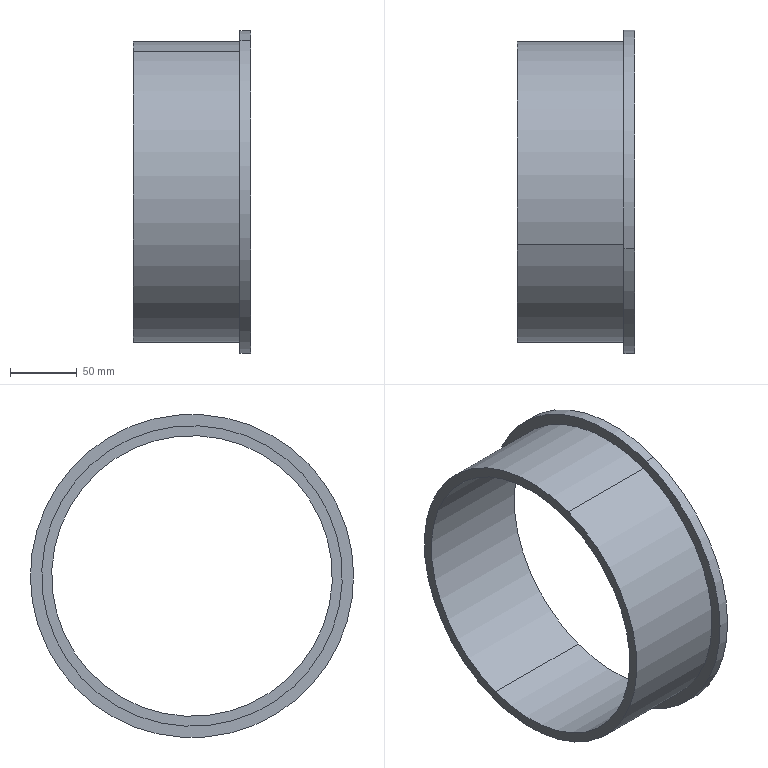Component | SolidWorks | AdjustingScrew-1 | 1 solid | 9 faces | box 88 x 243 x 243 mm | volume 503145 mm3 | cylinder 6 | plane 3 | commonest cylinder face diameters 226 x2 243 x2 211 x2
build123d program:
from build123d import *


with BuildPart() as part:
    # Sketch1 → Revolve1 (revolve)
    with BuildSketch(Plane.XY, mode=Mode.PRIVATE) as revolve1_sk:
        Polygon((0, 105.5), (88, 105.5), (88, 121.5), (80, 121.5), (80, 113), (0, 113), align=None)
    revolve(revolve1_sk.sketch.rotate(Axis((0, 0, 0), (1, 0, 0)), 90), axis=Axis((0, 0, 0), (1, 0, 0)))


solid = part.part

# Placed as in the assembly
solid = solid.moved(Location((-126, 0, 0), (0, 0, 0)))
STEP:
#1=COLOUR_RGB('',0.7922,0.8196,0.9333);
#2=FILL_AREA_STYLE_COLOUR('',#1);
#3=FILL_AREA_STYLE('',(#2));
#4=SURFACE_STYLE_FILL_AREA(#3);
#5=SURFACE_SIDE_STYLE('',(#4));
#6=SURFACE_STYLE_USAGE(.BOTH.,#5);
#7=PRESENTATION_STYLE_ASSIGNMENT((#6));
#8=CARTESIAN_POINT('',(-1.811,-1.573,4.161));
#9=VERTEX_POINT('',#8);
#10=CARTESIAN_POINT('',(-1.811,1.573,-4.161));
#11=VERTEX_POINT('',#10);
#12=CARTESIAN_POINT('',(-1.811,-0.,0.));
#13=DIRECTION('',(-1.,-0.,0.));
#14=DIRECTION('',(0.,-0.3537,0.9354));
#15=AXIS2_PLACEMENT_3D('',#12,#13,#14);
#16=CIRCLE('',#15,4.449);
#17=EDGE_CURVE('',#9,#11,#16,.T.);
#18=ORIENTED_EDGE('',*,*,#17,.T.);
#19=CARTESIAN_POINT('',(-4.961,1.573,-4.161));
#20=VERTEX_POINT('',#19);
#21=CARTESIAN_POINT('',(-4.961,1.573,-4.161));
#22=DIRECTION('',(-1.,-0.,0.));
#23=VECTOR('',#22,39.37);
#24=LINE('',#21,#23);
#25=EDGE_CURVE('',#11,#20,#24,.T.);
#26=ORIENTED_EDGE('',*,*,#25,.T.);
#27=CARTESIAN_POINT('',(-4.961,-1.573,4.161));
#28=VERTEX_POINT('',#27);
#29=CARTESIAN_POINT('',(-4.961,-0.,0.));
#30=DIRECTION('',(-1.,-0.,0.));
#31=DIRECTION('',(0.,-0.3537,0.9354));
#32=AXIS2_PLACEMENT_3D('',#29,#30,#31);
#33=CIRCLE('',#32,4.449);
#34=EDGE_CURVE('',#28,#20,#33,.T.);
#35=ORIENTED_EDGE('',*,*,#34,.F.);
#36=CARTESIAN_POINT('',(-4.961,-1.573,4.161));
#37=DIRECTION('',(-1.,-0.,0.));
#38=VECTOR('',#37,39.37);
#39=LINE('',#36,#38);
#40=EDGE_CURVE('',#9,#28,#39,.T.);
#41=ORIENTED_EDGE('',*,*,#40,.F.);
#42=EDGE_LOOP('',(#18,#26,#35,#41));
#43=FACE_OUTER_BOUND('',#42,.T.);
#44=CARTESIAN_POINT('',(-4.961,-0.,0.));
#45=DIRECTION('',(-1.,-0.,0.));
#46=DIRECTION('',(0.,-0.3537,0.9354));
#47=AXIS2_PLACEMENT_3D('',#44,#45,#46);
#48=CYLINDRICAL_SURFACE('',#47,4.449);
#49=ADVANCED_FACE('',(#43),#48,.T.);
#50=CARTESIAN_POINT('',(-1.496,-1.692,4.474));
#51=VERTEX_POINT('',#50);
#52=CARTESIAN_POINT('',(-1.496,1.692,-4.474));
#53=VERTEX_POINT('',#52);
#54=CARTESIAN_POINT('',(-1.496,-0.,0.));
#55=DIRECTION('',(-1.,-0.,0.));
#56=DIRECTION('',(0.,-0.3537,0.9354));
#57=AXIS2_PLACEMENT_3D('',#54,#55,#56);
#58=CIRCLE('',#57,4.783);
#59=EDGE_CURVE('',#51,#53,#58,.T.);
#60=ORIENTED_EDGE('',*,*,#59,.T.);
#61=CARTESIAN_POINT('',(-1.811,1.692,-4.474));
#62=VERTEX_POINT('',#61);
#63=CARTESIAN_POINT('',(-4.961,1.692,-4.474));
#64=DIRECTION('',(-1.,-0.,0.));
#65=VECTOR('',#64,39.37);
#66=LINE('',#63,#65);
#67=EDGE_CURVE('',#53,#62,#66,.T.);
#68=ORIENTED_EDGE('',*,*,#67,.T.);
#69=CARTESIAN_POINT('',(-1.811,-1.692,4.474));
#70=VERTEX_POINT('',#69);
#71=CARTESIAN_POINT('',(-1.811,-0.,0.));
#72=DIRECTION('',(-1.,-0.,0.));
#73=DIRECTION('',(0.,-0.3537,0.9354));
#74=AXIS2_PLACEMENT_3D('',#71,#72,#73);
#75=CIRCLE('',#74,4.783);
#76=EDGE_CURVE('',#70,#62,#75,.T.);
#77=ORIENTED_EDGE('',*,*,#76,.F.);
#78=CARTESIAN_POINT('',(-4.961,-1.692,4.474));
#79=DIRECTION('',(-1.,-0.,0.));
#80=VECTOR('',#79,39.37);
#81=LINE('',#78,#80);
#82=EDGE_CURVE('',#51,#70,#81,.T.);
#83=ORIENTED_EDGE('',*,*,#82,.F.);
#84=EDGE_LOOP('',(#60,#68,#77,#83));
#85=FACE_OUTER_BOUND('',#84,.T.);
#86=CARTESIAN_POINT('',(-4.961,-0.,0.));
#87=DIRECTION('',(-1.,-0.,0.));
#88=DIRECTION('',(0.,-0.3537,0.9354));
#89=AXIS2_PLACEMENT_3D('',#86,#87,#88);
#90=CYLINDRICAL_SURFACE('',#89,4.783);
#91=ADVANCED_FACE('',(#85),#90,.T.);
#92=CARTESIAN_POINT('',(-1.496,1.469,-3.885));
#93=VERTEX_POINT('',#92);
#94=CARTESIAN_POINT('',(-1.496,-1.469,3.885));
#95=VERTEX_POINT('',#94);
#96=CARTESIAN_POINT('',(-1.496,-0.,0.));
#97=DIRECTION('',(-1.,-0.,0.));
#98=DIRECTION('',(0.,-0.3537,0.9354));
#99=AXIS2_PLACEMENT_3D('',#96,#97,#98);
#100=CIRCLE('',#99,4.154);
#101=EDGE_CURVE('',#93,#95,#100,.T.);
#102=ORIENTED_EDGE('',*,*,#101,.F.);
#103=CARTESIAN_POINT('',(-4.961,1.469,-3.885));
#104=VERTEX_POINT('',#103);
#105=CARTESIAN_POINT('',(-4.961,1.469,-3.885));
#106=DIRECTION('',(-1.,-0.,0.));
#107=VECTOR('',#106,39.37);
#108=LINE('',#105,#107);
#109=EDGE_CURVE('',#93,#104,#108,.T.);
#110=ORIENTED_EDGE('',*,*,#109,.T.);
#111=CARTESIAN_POINT('',(-4.961,-1.469,3.885));
#112=VERTEX_POINT('',#111);
#113=CARTESIAN_POINT('',(-4.961,-0.,0.));
#114=DIRECTION('',(-1.,-0.,0.));
#115=DIRECTION('',(0.,-0.3537,0.9354));
#116=AXIS2_PLACEMENT_3D('',#113,#114,#115);
#117=CIRCLE('',#116,4.154);
#118=EDGE_CURVE('',#104,#112,#117,.T.);
#119=ORIENTED_EDGE('',*,*,#118,.T.);
#120=CARTESIAN_POINT('',(-4.961,-1.469,3.885));
#121=DIRECTION('',(-1.,-0.,0.));
#122=VECTOR('',#121,39.37);
#123=LINE('',#120,#122);
#124=EDGE_CURVE('',#95,#112,#123,.T.);
#125=ORIENTED_EDGE('',*,*,#124,.F.);
#126=EDGE_LOOP('',(#102,#110,#119,#125));
#127=FACE_OUTER_BOUND('',#126,.T.);
#128=CARTESIAN_POINT('',(-4.961,-0.,0.));
#129=DIRECTION('',(-1.,-0.,0.));
#130=DIRECTION('',(0.,-0.3537,0.9354));
#131=AXIS2_PLACEMENT_3D('',#128,#129,#130);
#132=CYLINDRICAL_SURFACE('',#131,4.154);
#133=ADVANCED_FACE('',(#127),#132,.F.);
#134=CARTESIAN_POINT('',(-4.961,-0.,0.));
#135=DIRECTION('',(-1.,-0.,0.));
#136=DIRECTION('',(0.,-0.3537,0.9354));
#137=AXIS2_PLACEMENT_3D('',#134,#135,#136);
#138=CIRCLE('',#137,4.154);
#139=EDGE_CURVE('',#112,#104,#138,.T.);
#140=ORIENTED_EDGE('',*,*,#139,.F.);
#141=ORIENTED_EDGE('',*,*,#118,.F.);
#142=EDGE_LOOP('',(#140,#141));
#143=FACE_BOUND('',#142,.T.);
#144=ORIENTED_EDGE('',*,*,#34,.T.);
#145=CARTESIAN_POINT('',(-4.961,-0.,0.));
#146=DIRECTION('',(-1.,-0.,0.));
#147=DIRECTION('',(0.,-0.3537,0.9354));
#148=AXIS2_PLACEMENT_3D('',#145,#146,#147);
#149=CIRCLE('',#148,4.449);
#150=EDGE_CURVE('',#20,#28,#149,.T.);
#151=ORIENTED_EDGE('',*,*,#150,.T.);
#152=EDGE_LOOP('',(#144,#151));
#153=FACE_OUTER_BOUND('',#152,.T.);
#154=CARTESIAN_POINT('',(-4.961,4.161,1.573));
#155=DIRECTION('',(1.,0.,-0.));
#156=DIRECTION('',(-0.,0.3537,-0.9354));
#157=AXIS2_PLACEMENT_3D('',#154,#155,#156);
#158=PLANE('',#157);
#159=ADVANCED_FACE('',(#143,#153),#158,.F.);
#160=ORIENTED_EDGE('',*,*,#109,.F.);
#161=CARTESIAN_POINT('',(-1.496,-0.,0.));
#162=DIRECTION('',(-1.,-0.,0.));
#163=DIRECTION('',(0.,-0.3537,0.9354));
#164=AXIS2_PLACEMENT_3D('',#161,#162,#163);
#165=CIRCLE('',#164,4.154);
#166=EDGE_CURVE('',#95,#93,#165,.T.);
#167=ORIENTED_EDGE('',*,*,#166,.F.);
#168=ORIENTED_EDGE('',*,*,#124,.T.);
#169=ORIENTED_EDGE('',*,*,#139,.T.);
#170=EDGE_LOOP('',(#160,#167,#168,#169));
#171=FACE_OUTER_BOUND('',#170,.T.);
#172=CARTESIAN_POINT('',(-4.961,-0.,0.));
#173=DIRECTION('',(-1.,-0.,0.));
#174=DIRECTION('',(0.,-0.3537,0.9354));
#175=AXIS2_PLACEMENT_3D('',#172,#173,#174);
#176=CYLINDRICAL_SURFACE('',#175,4.154);
#177=ADVANCED_FACE('',(#171),#176,.F.);
#178=ORIENTED_EDGE('',*,*,#59,.F.);
#179=CARTESIAN_POINT('',(-1.496,-0.,0.));
#180=DIRECTION('',(-1.,-0.,0.));
#181=DIRECTION('',(0.,-0.3537,0.9354));
#182=AXIS2_PLACEMENT_3D('',#179,#180,#181);
#183=CIRCLE('',#182,4.783);
#184=EDGE_CURVE('',#53,#51,#183,.T.);
#185=ORIENTED_EDGE('',*,*,#184,.F.);
#186=EDGE_LOOP('',(#178,#185));
#187=FACE_OUTER_BOUND('',#186,.T.);
#188=ORIENTED_EDGE('',*,*,#166,.T.);
#189=ORIENTED_EDGE('',*,*,#101,.T.);
#190=EDGE_LOOP('',(#188,#189));
#191=FACE_BOUND('',#190,.T.);
#192=CARTESIAN_POINT('',(-1.496,3.885,1.469));
#193=DIRECTION('',(-1.,-0.,0.));
#194=DIRECTION('',(0.,-0.3537,0.9354));
#195=AXIS2_PLACEMENT_3D('',#192,#193,#194);
#196=PLANE('',#195);
#197=ADVANCED_FACE('',(#187,#191),#196,.F.);
#198=ORIENTED_EDGE('',*,*,#67,.F.);
#199=ORIENTED_EDGE('',*,*,#184,.T.);
#200=ORIENTED_EDGE('',*,*,#82,.T.);
#201=CARTESIAN_POINT('',(-1.811,-0.,0.));
#202=DIRECTION('',(-1.,-0.,0.));
#203=DIRECTION('',(0.,-0.3537,0.9354));
#204=AXIS2_PLACEMENT_3D('',#201,#202,#203);
#205=CIRCLE('',#204,4.783);
#206=EDGE_CURVE('',#62,#70,#205,.T.);
#207=ORIENTED_EDGE('',*,*,#206,.F.);
#208=EDGE_LOOP('',(#198,#199,#200,#207));
#209=FACE_OUTER_BOUND('',#208,.T.);
#210=CARTESIAN_POINT('',(-4.961,-0.,0.));
#211=DIRECTION('',(-1.,-0.,0.));
#212=DIRECTION('',(0.,-0.3537,0.9354));
#213=AXIS2_PLACEMENT_3D('',#210,#211,#212);
#214=CYLINDRICAL_SURFACE('',#213,4.783);
#215=ADVANCED_FACE('',(#209),#214,.T.);
#216=ORIENTED_EDGE('',*,*,#17,.F.);
#217=CARTESIAN_POINT('',(-1.811,-0.,0.));
#218=DIRECTION('',(-1.,-0.,0.));
#219=DIRECTION('',(0.,-0.3537,0.9354));
#220=AXIS2_PLACEMENT_3D('',#217,#218,#219);
#221=CIRCLE('',#220,4.449);
#222=EDGE_CURVE('',#11,#9,#221,.T.);
#223=ORIENTED_EDGE('',*,*,#222,.F.);
#224=EDGE_LOOP('',(#216,#223));
#225=FACE_BOUND('',#224,.T.);
#226=ORIENTED_EDGE('',*,*,#76,.T.);
#227=ORIENTED_EDGE('',*,*,#206,.T.);
#228=EDGE_LOOP('',(#226,#227));
#229=FACE_OUTER_BOUND('',#228,.T.);
#230=CARTESIAN_POINT('',(-1.811,4.474,1.692));
#231=DIRECTION('',(1.,0.,-0.));
#232=DIRECTION('',(-0.,0.3537,-0.9354));
#233=AXIS2_PLACEMENT_3D('',#230,#231,#232);
#234=PLANE('',#233);
#235=ADVANCED_FACE('',(#225,#229),#234,.F.);
#236=ORIENTED_EDGE('',*,*,#25,.F.);
#237=ORIENTED_EDGE('',*,*,#222,.T.);
#238=ORIENTED_EDGE('',*,*,#40,.T.);
#239=ORIENTED_EDGE('',*,*,#150,.F.);
#240=EDGE_LOOP('',(#236,#237,#238,#239));
#241=FACE_OUTER_BOUND('',#240,.T.);
#242=CARTESIAN_POINT('',(-4.961,-0.,0.));
#243=DIRECTION('',(-1.,-0.,0.));
#244=DIRECTION('',(0.,-0.3537,0.9354));
#245=AXIS2_PLACEMENT_3D('',#242,#243,#244);
#246=CYLINDRICAL_SURFACE('',#245,4.449);
#247=ADVANCED_FACE('',(#241),#246,.T.);
#248=CLOSED_SHELL('',(#49,#91,#133,#159,#177,#197,#215,#235,#247));
#249=MANIFOLD_SOLID_BREP('',#248);
#250=STYLED_ITEM('',(#7),#249);
#251=PRESENTATION_LAYER_ASSIGNMENT('','',(#250));
#252=CARTESIAN_POINT('',(0.,0.,0.));
#253=DIRECTION('',(0.,0.,1.));
#254=DIRECTION('',(1.,0.,0.));
#255=AXIS2_PLACEMENT_3D('',#252,#253,#254);
#256=(LENGTH_UNIT()NAMED_UNIT(*)SI_UNIT($,.METRE.));
#257=LENGTH_MEASURE_WITH_UNIT(LENGTH_MEASURE(0.0254),#256);
#258=DIMENSIONAL_EXPONENTS(1.,0.,0.,0.,0.,0.,0.);
#259=(CONVERSION_BASED_UNIT('',#257)LENGTH_UNIT()NAMED_UNIT(#258));
#260=UNCERTAINTY_MEASURE_WITH_UNIT(LENGTH_MEASURE(0.00001),#259,'','');
#261=(NAMED_UNIT(*)PLANE_ANGLE_UNIT()SI_UNIT($,.RADIAN.));
#262=(NAMED_UNIT(*)SI_UNIT($,.STERADIAN.)SOLID_ANGLE_UNIT());
#263=(GEOMETRIC_REPRESENTATION_CONTEXT(3)GLOBAL_UNCERTAINTY_ASSIGNED_CONTEXT((#260))GLOBAL_UNIT_ASSIGNED_CONTEXT((#259,#261,#262))REPRESENTATION_CONTEXT('',''));
#264=ADVANCED_BREP_SHAPE_REPRESENTATION('',(#249,#255),#263);
#265=(LENGTH_UNIT()NAMED_UNIT(*)SI_UNIT($,.METRE.));
#266=LENGTH_MEASURE_WITH_UNIT(LENGTH_MEASURE(0.0254),#265);
#267=DIMENSIONAL_EXPONENTS(1.,0.,0.,0.,0.,0.,0.);
#268=(CONVERSION_BASED_UNIT('',#266)LENGTH_UNIT()NAMED_UNIT(#267));
#269=UNCERTAINTY_MEASURE_WITH_UNIT(LENGTH_MEASURE(0.00001),#268,'','');
#270=(NAMED_UNIT(*)PLANE_ANGLE_UNIT()SI_UNIT($,.RADIAN.));
#271=(NAMED_UNIT(*)SI_UNIT($,.STERADIAN.)SOLID_ANGLE_UNIT());
#272=(GEOMETRIC_REPRESENTATION_CONTEXT(3)GLOBAL_UNCERTAINTY_ASSIGNED_CONTEXT((#269))GLOBAL_UNIT_ASSIGNED_CONTEXT((#268,#270,#271))REPRESENTATION_CONTEXT('',''));
#273=MECHANICAL_DESIGN_GEOMETRIC_PRESENTATION_REPRESENTATION('',(#250),#272);